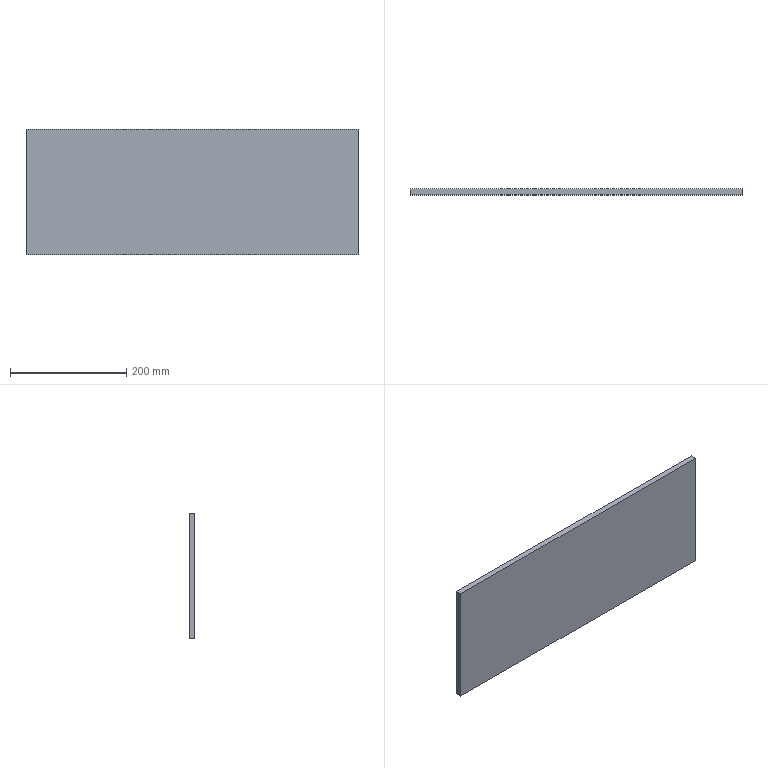Component | SolidWorks | PushPlate-1 | 1 solid | 6 faces | box 570 x 10 x 215 mm | volume 1225500 mm3 | plane 6
build123d program:
from build123d import *

# Parameters (mm, degrees)
SKETCH1_W           = 570
SKETCH1_H           = 215
BOSS_EXTRUDE1_DEPTH = 10


with BuildPart() as part:
    # Sketch1 → Boss-Extrude1 (new body)
    with BuildSketch(Plane.XY):
        Rectangle(SKETCH1_W, SKETCH1_H)
    extrude(amount=BOSS_EXTRUDE1_DEPTH)


solid = part.part

# Placed as in the assembly
solid = solid.moved(Location((25.629, -1206.787, 90.661), (90, 0, 0)))
STEP:
#1=COLOUR_RGB('',0.7922,0.8196,0.9333);
#2=FILL_AREA_STYLE_COLOUR('',#1);
#3=FILL_AREA_STYLE('',(#2));
#4=SURFACE_STYLE_FILL_AREA(#3);
#5=SURFACE_SIDE_STYLE('',(#4));
#6=SURFACE_STYLE_USAGE(.BOTH.,#5);
#7=PRESENTATION_STYLE_ASSIGNMENT((#6));
#8=CARTESIAN_POINT('',(12.23,-47.511,-0.663));
#9=VERTEX_POINT('',#8);
#10=CARTESIAN_POINT('',(12.23,-47.511,7.802));
#11=VERTEX_POINT('',#10);
#12=CARTESIAN_POINT('',(12.23,-47.511,-0.663));
#13=DIRECTION('',(-0.,0.,1.));
#14=VECTOR('',#13,39.37);
#15=LINE('',#12,#14);
#16=EDGE_CURVE('',#9,#11,#15,.T.);
#17=ORIENTED_EDGE('',*,*,#16,.T.);
#18=CARTESIAN_POINT('',(12.23,-47.905,7.802));
#19=VERTEX_POINT('',#18);
#20=CARTESIAN_POINT('',(12.23,-47.905,7.802));
#21=DIRECTION('',(-0.,1.,0.));
#22=VECTOR('',#21,39.37);
#23=LINE('',#20,#22);
#24=EDGE_CURVE('',#19,#11,#23,.T.);
#25=ORIENTED_EDGE('',*,*,#24,.F.);
#26=CARTESIAN_POINT('',(12.23,-47.905,-0.663));
#27=VERTEX_POINT('',#26);
#28=CARTESIAN_POINT('',(12.23,-47.905,-0.663));
#29=DIRECTION('',(-0.,0.,1.));
#30=VECTOR('',#29,39.37);
#31=LINE('',#28,#30);
#32=EDGE_CURVE('',#27,#19,#31,.T.);
#33=ORIENTED_EDGE('',*,*,#32,.F.);
#34=CARTESIAN_POINT('',(12.23,-47.905,-0.663));
#35=DIRECTION('',(-0.,1.,0.));
#36=VECTOR('',#35,39.37);
#37=LINE('',#34,#36);
#38=EDGE_CURVE('',#27,#9,#37,.T.);
#39=ORIENTED_EDGE('',*,*,#38,.T.);
#40=EDGE_LOOP('',(#17,#25,#33,#39));
#41=FACE_OUTER_BOUND('',#40,.T.);
#42=CARTESIAN_POINT('',(12.23,-47.905,-0.663));
#43=DIRECTION('',(-1.,-0.,-0.));
#44=DIRECTION('',(0.,-1.,-0.));
#45=AXIS2_PLACEMENT_3D('',#42,#43,#44);
#46=PLANE('',#45);
#47=ADVANCED_FACE('',(#41),#46,.F.);
#48=CARTESIAN_POINT('',(-10.211,-47.511,7.802));
#49=VERTEX_POINT('',#48);
#50=CARTESIAN_POINT('',(-10.211,-47.511,7.802));
#51=DIRECTION('',(-1.,-0.,-0.));
#52=VECTOR('',#51,39.37);
#53=LINE('',#50,#52);
#54=EDGE_CURVE('',#11,#49,#53,.T.);
#55=ORIENTED_EDGE('',*,*,#54,.T.);
#56=CARTESIAN_POINT('',(-10.211,-47.905,7.802));
#57=VERTEX_POINT('',#56);
#58=CARTESIAN_POINT('',(-10.211,-47.905,7.802));
#59=DIRECTION('',(-0.,1.,0.));
#60=VECTOR('',#59,39.37);
#61=LINE('',#58,#60);
#62=EDGE_CURVE('',#57,#49,#61,.T.);
#63=ORIENTED_EDGE('',*,*,#62,.F.);
#64=CARTESIAN_POINT('',(-10.211,-47.905,7.802));
#65=DIRECTION('',(-1.,-0.,-0.));
#66=VECTOR('',#65,39.37);
#67=LINE('',#64,#66);
#68=EDGE_CURVE('',#19,#57,#67,.T.);
#69=ORIENTED_EDGE('',*,*,#68,.F.);
#70=ORIENTED_EDGE('',*,*,#24,.T.);
#71=EDGE_LOOP('',(#55,#63,#69,#70));
#72=FACE_OUTER_BOUND('',#71,.T.);
#73=CARTESIAN_POINT('',(-10.211,-47.905,7.802));
#74=DIRECTION('',(0.,0.,-1.));
#75=DIRECTION('',(-0.,1.,0.));
#76=AXIS2_PLACEMENT_3D('',#73,#74,#75);
#77=PLANE('',#76);
#78=ADVANCED_FACE('',(#72),#77,.F.);
#79=CARTESIAN_POINT('',(-10.211,-47.511,-0.663));
#80=VERTEX_POINT('',#79);
#81=CARTESIAN_POINT('',(-10.211,-47.511,-0.663));
#82=DIRECTION('',(0.,-0.,-1.));
#83=VECTOR('',#82,39.37);
#84=LINE('',#81,#83);
#85=EDGE_CURVE('',#49,#80,#84,.T.);
#86=ORIENTED_EDGE('',*,*,#85,.T.);
#87=CARTESIAN_POINT('',(-10.211,-47.905,-0.663));
#88=VERTEX_POINT('',#87);
#89=CARTESIAN_POINT('',(-10.211,-47.905,-0.663));
#90=DIRECTION('',(-0.,1.,0.));
#91=VECTOR('',#90,39.37);
#92=LINE('',#89,#91);
#93=EDGE_CURVE('',#88,#80,#92,.T.);
#94=ORIENTED_EDGE('',*,*,#93,.F.);
#95=CARTESIAN_POINT('',(-10.211,-47.905,-0.663));
#96=DIRECTION('',(0.,-0.,-1.));
#97=VECTOR('',#96,39.37);
#98=LINE('',#95,#97);
#99=EDGE_CURVE('',#57,#88,#98,.T.);
#100=ORIENTED_EDGE('',*,*,#99,.F.);
#101=ORIENTED_EDGE('',*,*,#62,.T.);
#102=EDGE_LOOP('',(#86,#94,#100,#101));
#103=FACE_OUTER_BOUND('',#102,.T.);
#104=CARTESIAN_POINT('',(-10.211,-47.905,-0.663));
#105=DIRECTION('',(1.,0.,0.));
#106=DIRECTION('',(-0.,1.,0.));
#107=AXIS2_PLACEMENT_3D('',#104,#105,#106);
#108=PLANE('',#107);
#109=ADVANCED_FACE('',(#103),#108,.F.);
#110=CARTESIAN_POINT('',(-10.211,-47.511,-0.663));
#111=DIRECTION('',(1.,0.,0.));
#112=VECTOR('',#111,39.37);
#113=LINE('',#110,#112);
#114=EDGE_CURVE('',#80,#9,#113,.T.);
#115=ORIENTED_EDGE('',*,*,#114,.T.);
#116=ORIENTED_EDGE('',*,*,#38,.F.);
#117=CARTESIAN_POINT('',(-10.211,-47.905,-0.663));
#118=DIRECTION('',(1.,0.,0.));
#119=VECTOR('',#118,39.37);
#120=LINE('',#117,#119);
#121=EDGE_CURVE('',#88,#27,#120,.T.);
#122=ORIENTED_EDGE('',*,*,#121,.F.);
#123=ORIENTED_EDGE('',*,*,#93,.T.);
#124=EDGE_LOOP('',(#115,#116,#122,#123));
#125=FACE_OUTER_BOUND('',#124,.T.);
#126=CARTESIAN_POINT('',(-10.211,-47.905,-0.663));
#127=DIRECTION('',(-0.,-0.,1.));
#128=DIRECTION('',(0.,-1.,-0.));
#129=AXIS2_PLACEMENT_3D('',#126,#127,#128);
#130=PLANE('',#129);
#131=ADVANCED_FACE('',(#125),#130,.F.);
#132=ORIENTED_EDGE('',*,*,#32,.T.);
#133=ORIENTED_EDGE('',*,*,#68,.T.);
#134=ORIENTED_EDGE('',*,*,#99,.T.);
#135=ORIENTED_EDGE('',*,*,#121,.T.);
#136=EDGE_LOOP('',(#132,#133,#134,#135));
#137=FACE_OUTER_BOUND('',#136,.T.);
#138=CARTESIAN_POINT('',(1.009,-47.905,3.569));
#139=DIRECTION('',(-0.,1.,0.));
#140=DIRECTION('',(-1.,-0.,-0.));
#141=AXIS2_PLACEMENT_3D('',#138,#139,#140);
#142=PLANE('',#141);
#143=ADVANCED_FACE('',(#137),#142,.F.);
#144=ORIENTED_EDGE('',*,*,#16,.F.);
#145=ORIENTED_EDGE('',*,*,#114,.F.);
#146=ORIENTED_EDGE('',*,*,#85,.F.);
#147=ORIENTED_EDGE('',*,*,#54,.F.);
#148=EDGE_LOOP('',(#144,#145,#146,#147));
#149=FACE_OUTER_BOUND('',#148,.T.);
#150=CARTESIAN_POINT('',(1.009,-47.511,3.569));
#151=DIRECTION('',(-0.,1.,0.));
#152=DIRECTION('',(-1.,-0.,-0.));
#153=AXIS2_PLACEMENT_3D('',#150,#151,#152);
#154=PLANE('',#153);
#155=ADVANCED_FACE('',(#149),#154,.T.);
#156=CLOSED_SHELL('',(#47,#78,#109,#131,#143,#155));
#157=MANIFOLD_SOLID_BREP('',#156);
#158=STYLED_ITEM('',(#7),#157);
#159=PRESENTATION_LAYER_ASSIGNMENT('','',(#158));
#160=(LENGTH_UNIT()NAMED_UNIT(*)SI_UNIT($,.METRE.));
#161=LENGTH_MEASURE_WITH_UNIT(LENGTH_MEASURE(0.0254),#160);
#162=DIMENSIONAL_EXPONENTS(1.,0.,0.,0.,0.,0.,0.);
#163=(CONVERSION_BASED_UNIT('',#161)LENGTH_UNIT()NAMED_UNIT(#162));
#164=UNCERTAINTY_MEASURE_WITH_UNIT(LENGTH_MEASURE(0.00001),#163,'','');
#165=(NAMED_UNIT(*)PLANE_ANGLE_UNIT()SI_UNIT($,.RADIAN.));
#166=(NAMED_UNIT(*)SI_UNIT($,.STERADIAN.)SOLID_ANGLE_UNIT());
#167=(GEOMETRIC_REPRESENTATION_CONTEXT(3)GLOBAL_UNCERTAINTY_ASSIGNED_CONTEXT((#164))GLOBAL_UNIT_ASSIGNED_CONTEXT((#163,#165,#166))REPRESENTATION_CONTEXT('',''));
#168=MECHANICAL_DESIGN_GEOMETRIC_PRESENTATION_REPRESENTATION('',(#158),#167);
#169=CARTESIAN_POINT('',(0.,0.,0.));
#170=DIRECTION('',(0.,0.,1.));
#171=DIRECTION('',(1.,0.,0.));
#172=AXIS2_PLACEMENT_3D('',#169,#170,#171);
#173=(LENGTH_UNIT()NAMED_UNIT(*)SI_UNIT($,.METRE.));
#174=LENGTH_MEASURE_WITH_UNIT(LENGTH_MEASURE(0.0254),#173);
#175=DIMENSIONAL_EXPONENTS(1.,0.,0.,0.,0.,0.,0.);
#176=(CONVERSION_BASED_UNIT('',#174)LENGTH_UNIT()NAMED_UNIT(#175));
#177=UNCERTAINTY_MEASURE_WITH_UNIT(LENGTH_MEASURE(0.00001),#176,'','');
#178=(NAMED_UNIT(*)PLANE_ANGLE_UNIT()SI_UNIT($,.RADIAN.));
#179=(NAMED_UNIT(*)SI_UNIT($,.STERADIAN.)SOLID_ANGLE_UNIT());
#180=(GEOMETRIC_REPRESENTATION_CONTEXT(3)GLOBAL_UNCERTAINTY_ASSIGNED_CONTEXT((#177))GLOBAL_UNIT_ASSIGNED_CONTEXT((#176,#178,#179))REPRESENTATION_CONTEXT('',''));
#181=ADVANCED_BREP_SHAPE_REPRESENTATION('',(#157,#172),#180);